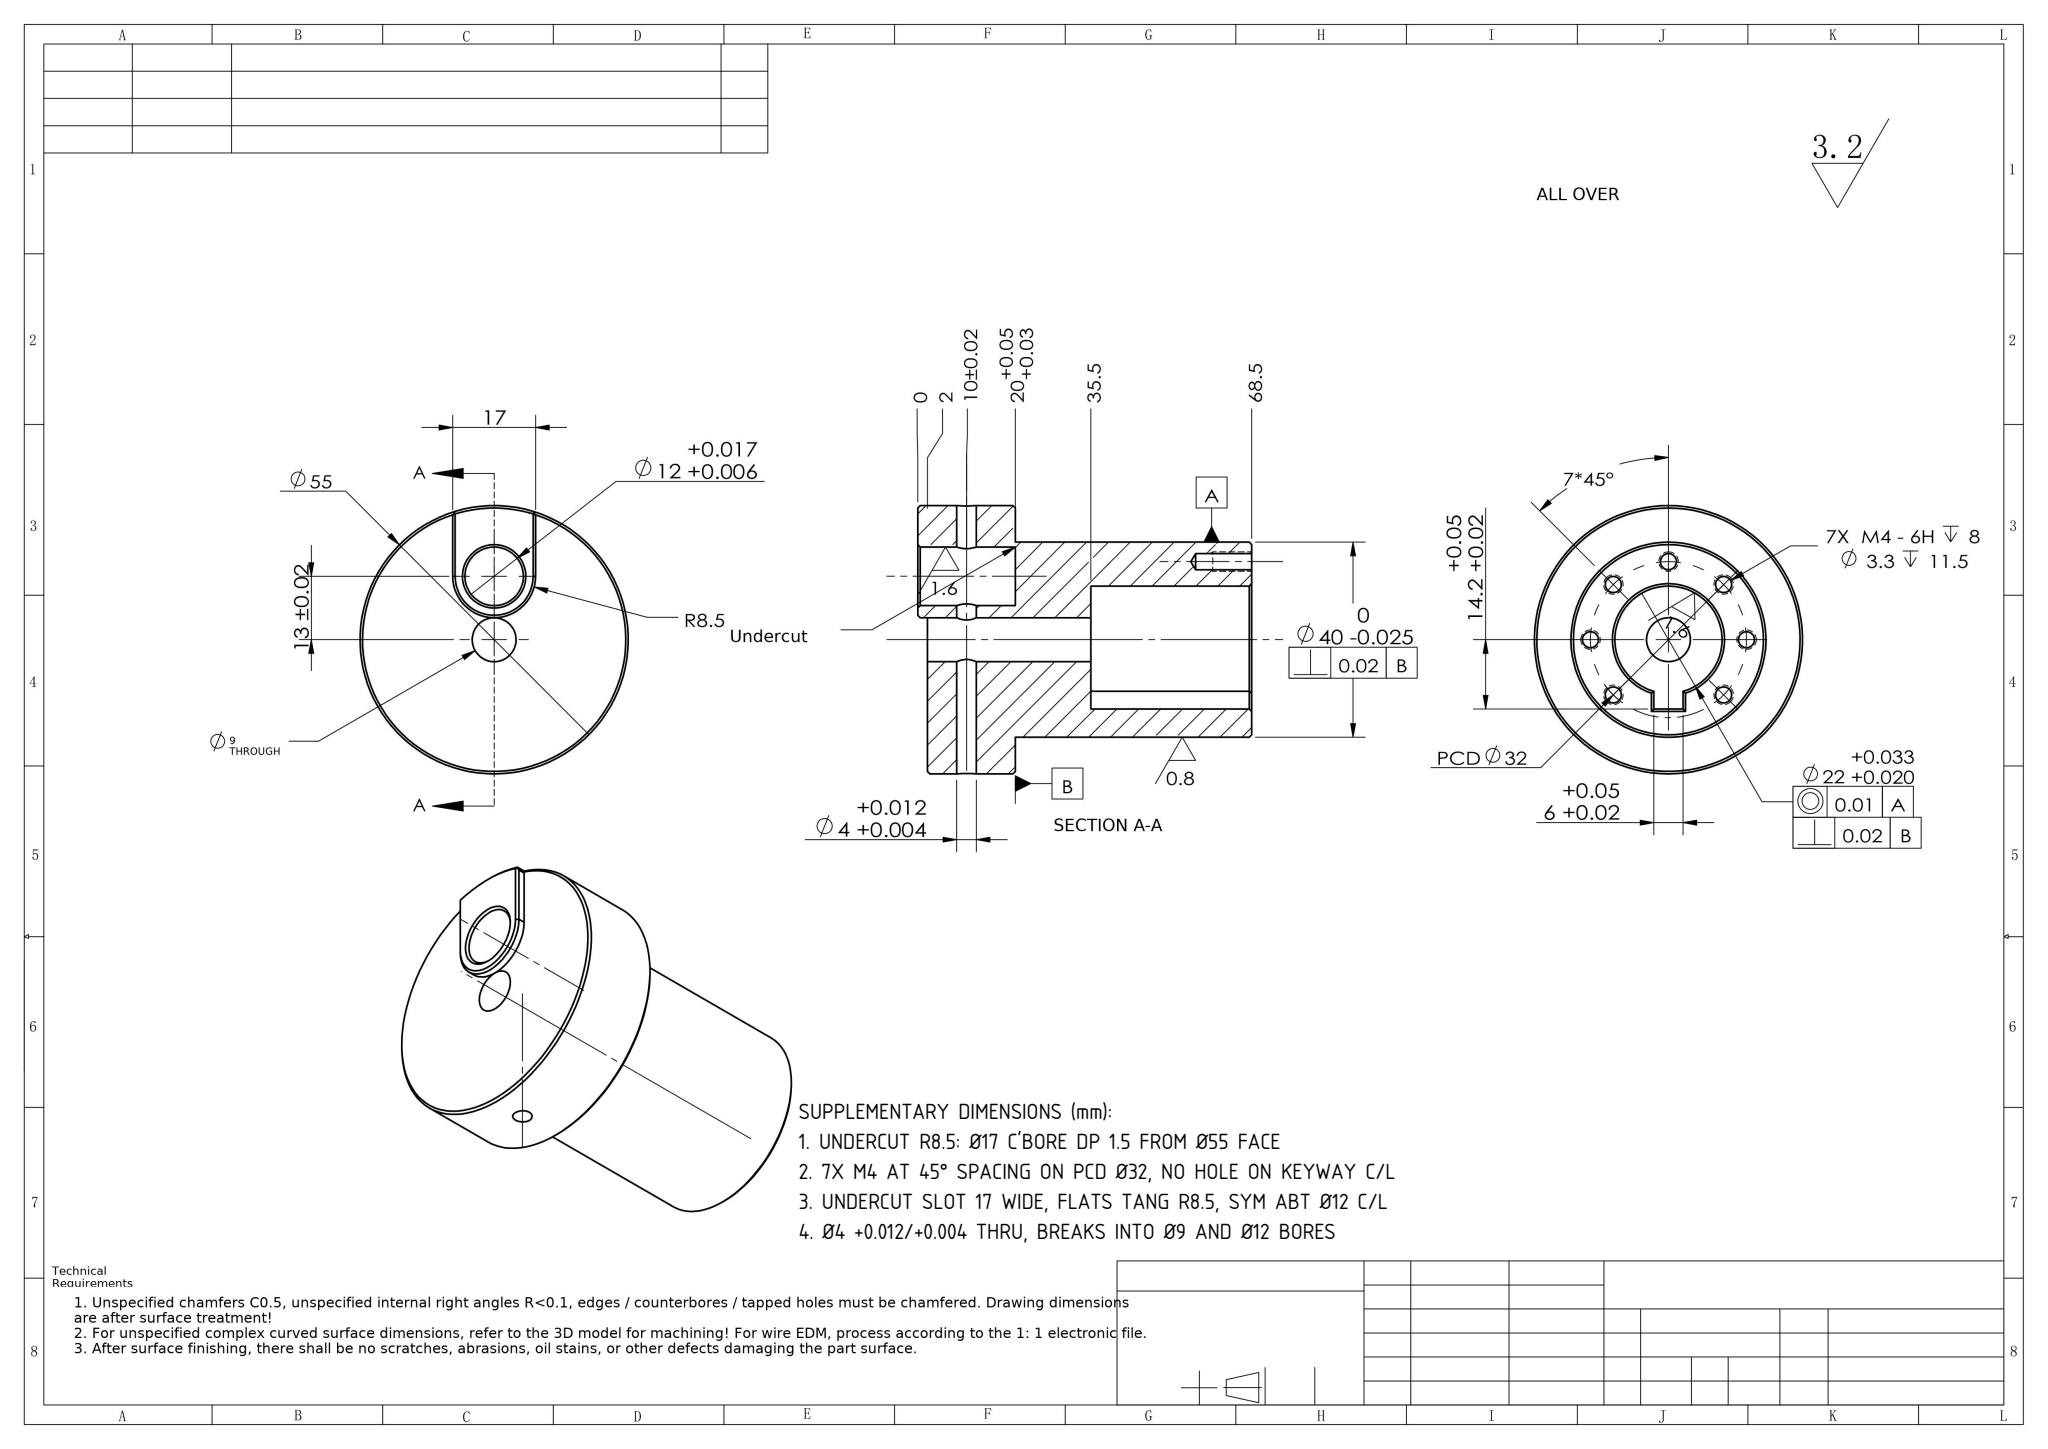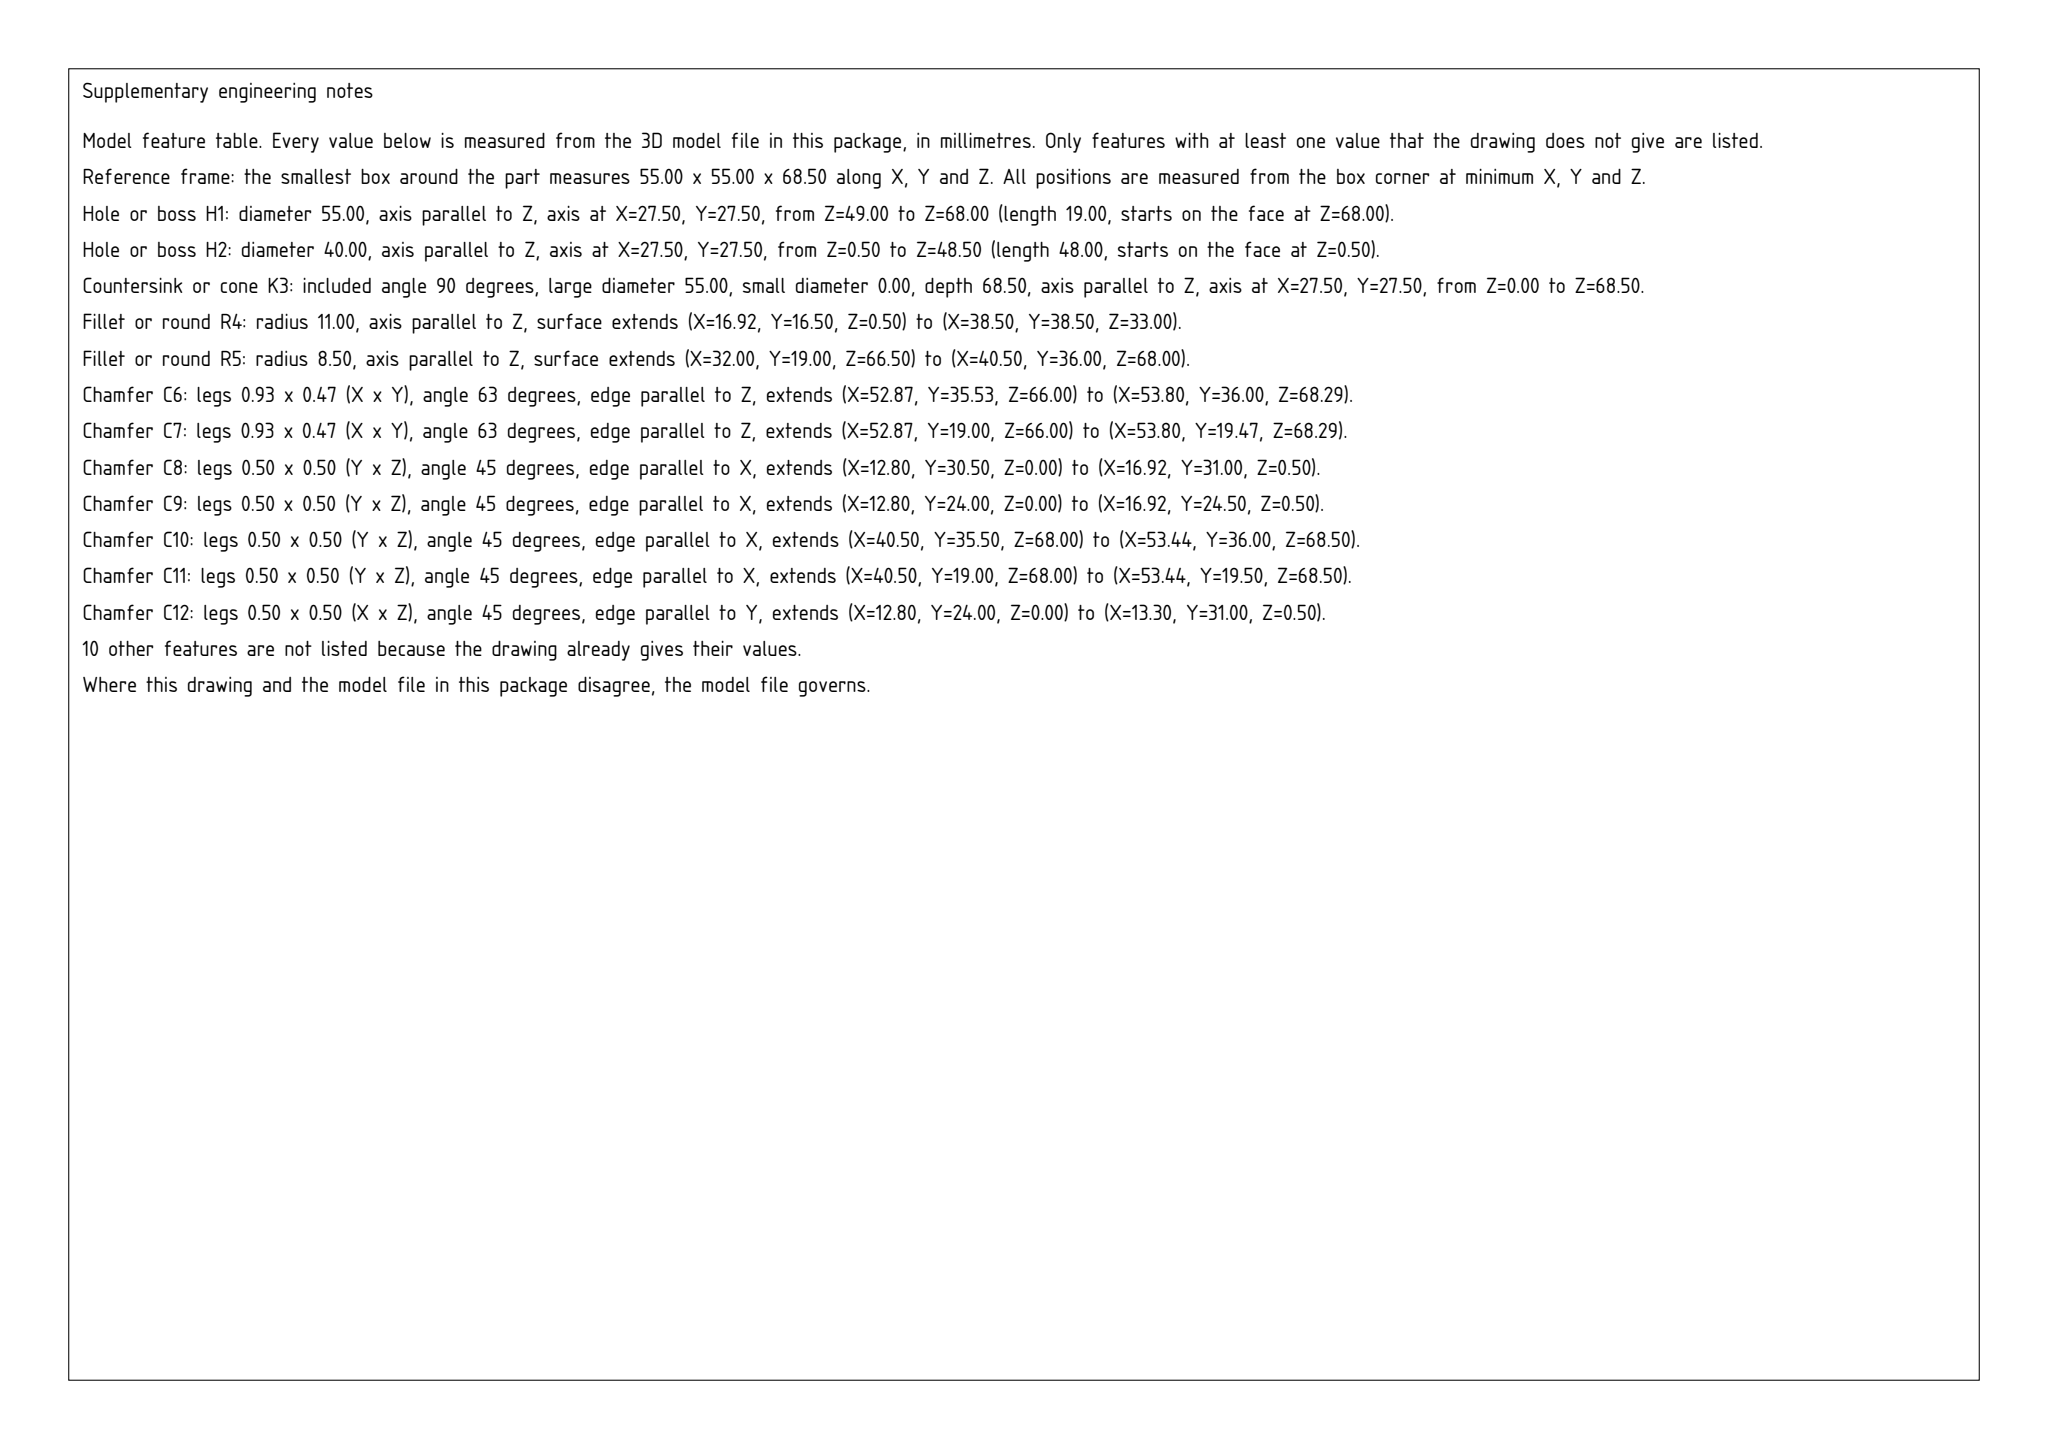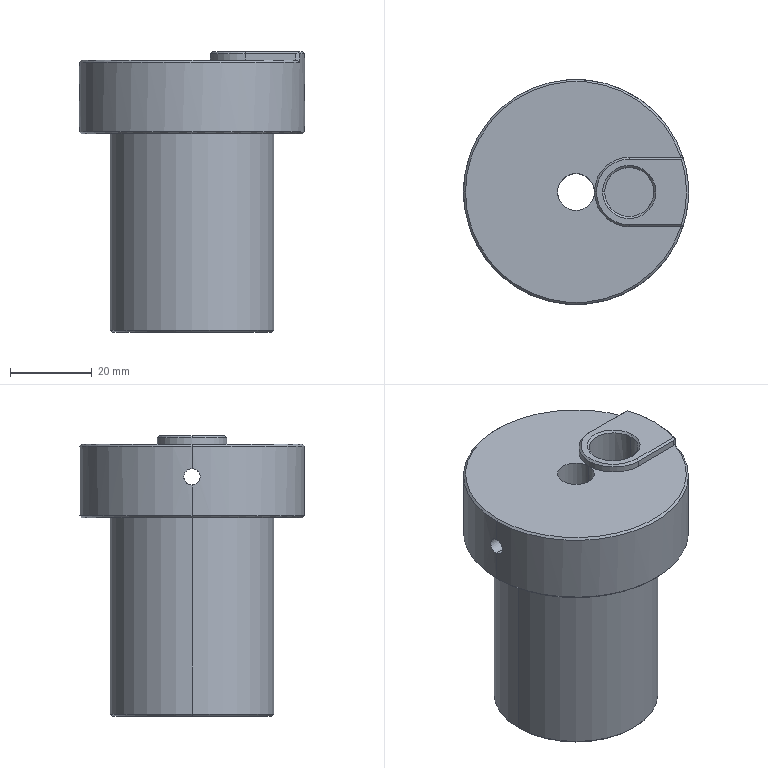Part | SolidWorks | mm | 1 solid | 74 faces | box 55 x 55 x 68.5 mm | volume 85598 mm3 | cylinder 30 | cone 26 | plane 18 | commonest cylinder face diameters 3.3 x14 4 x6 12 x2 40 x2 9 x2 55 x2 22 x1 17 x1